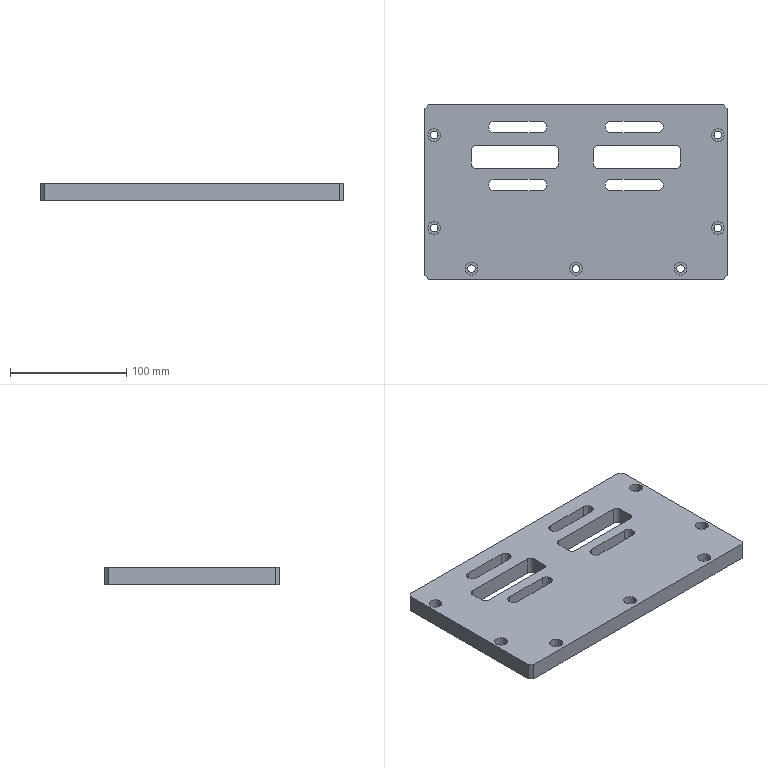Part | SolidWorks | mm | 1 solid | 81 faces | box 260 x 150 x 15 mm | volume 504942 mm3 | cylinder 48 | plane 33 | commonest cylinder face diameters 11 x14 6.6 x14 10 x12 8 x8